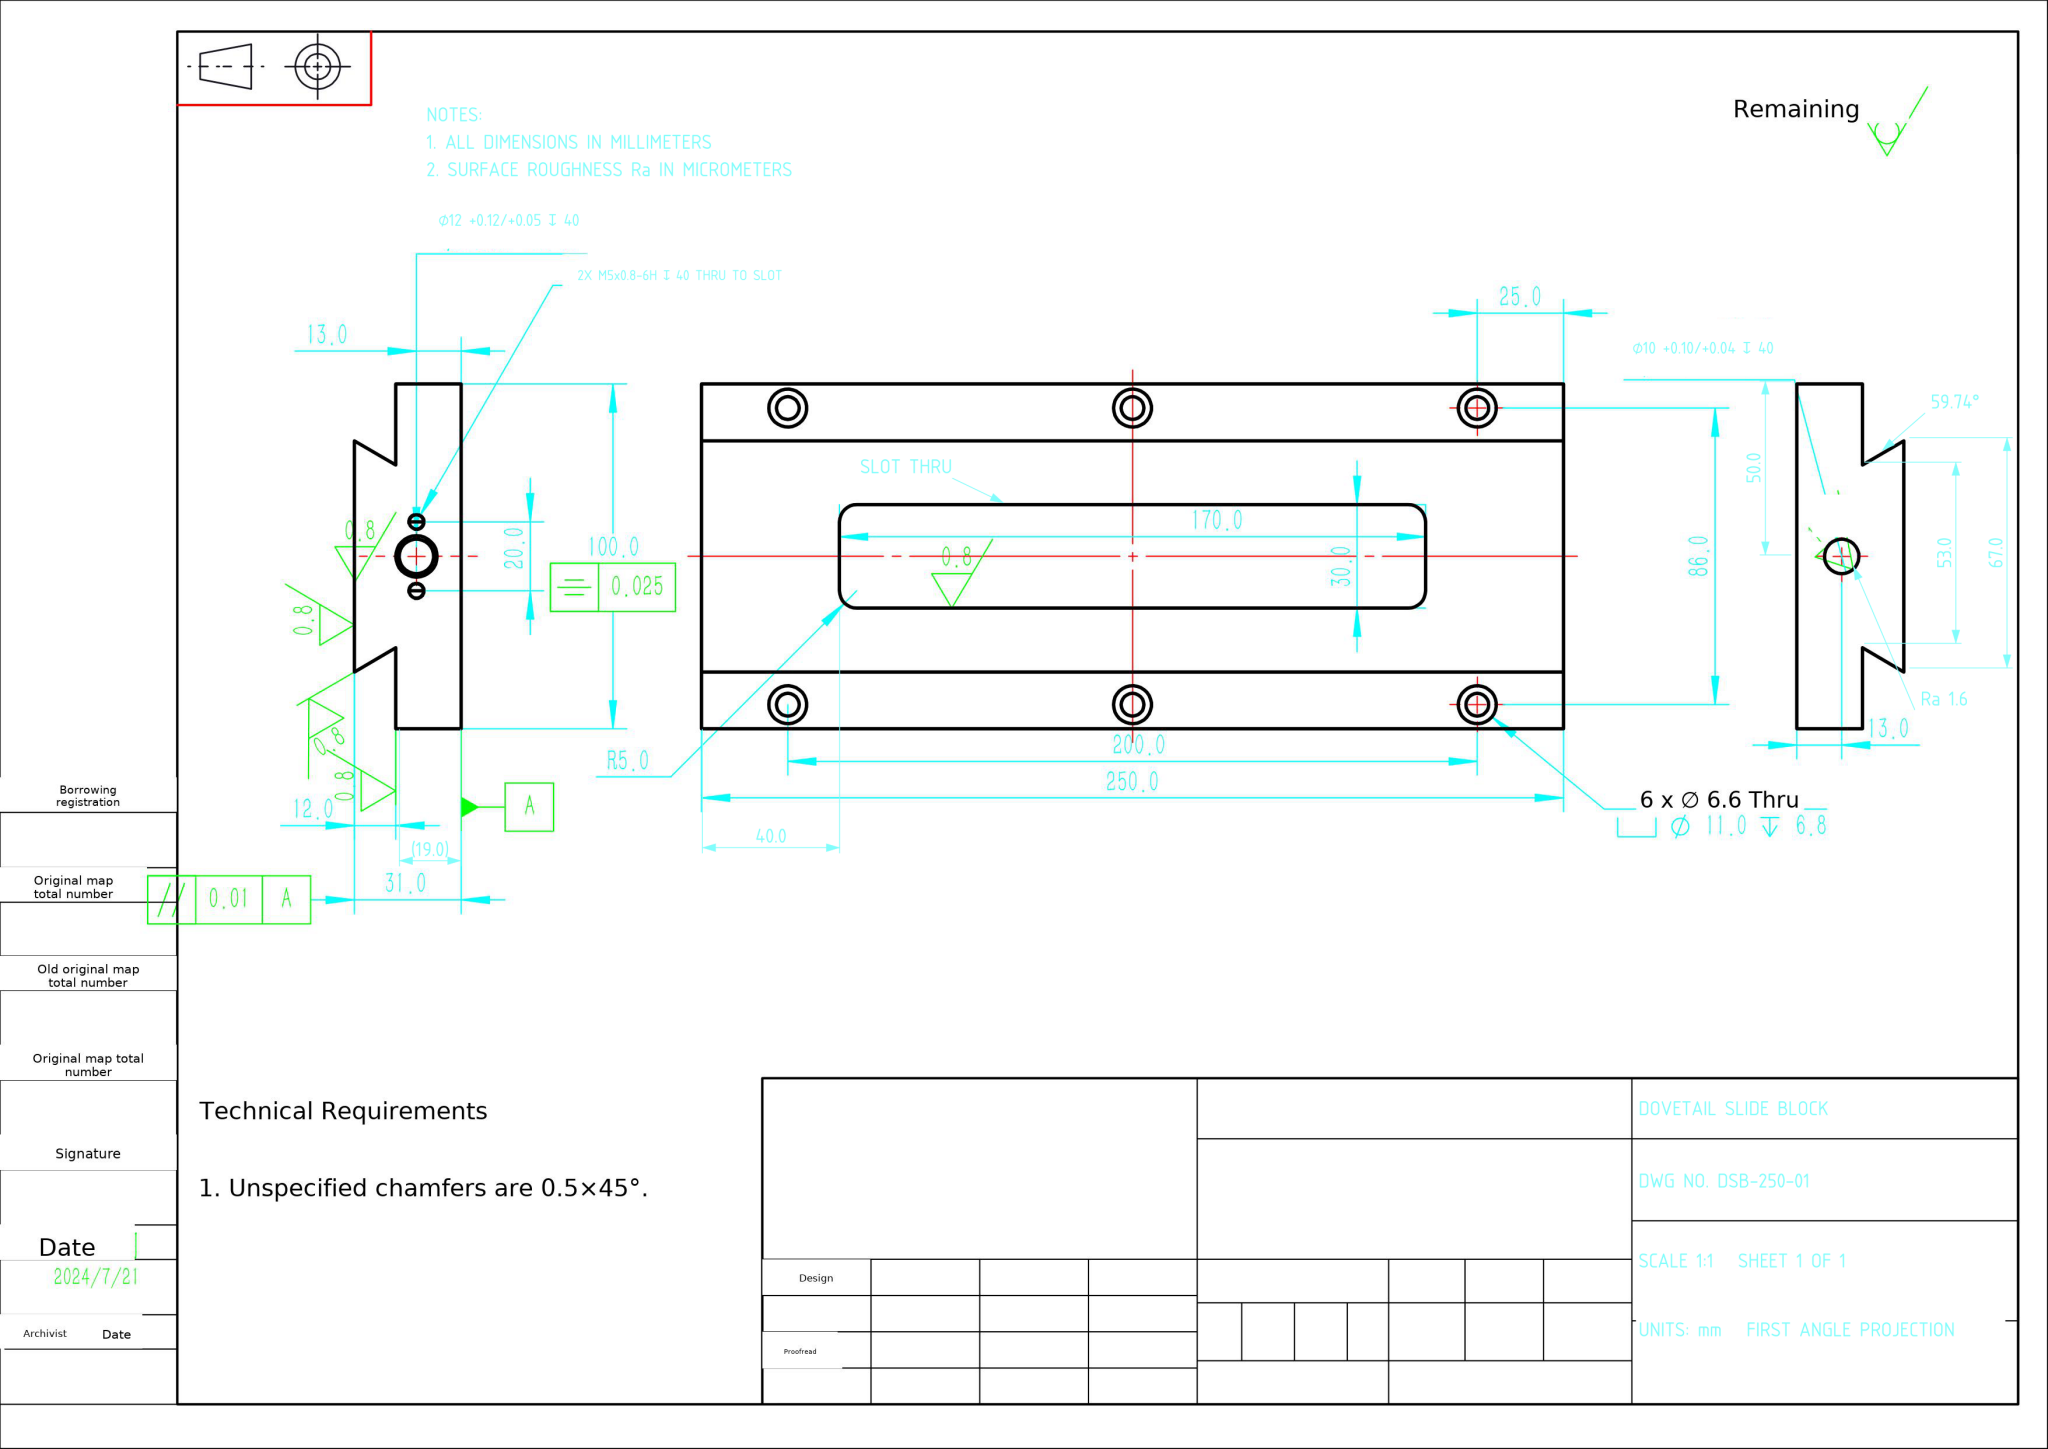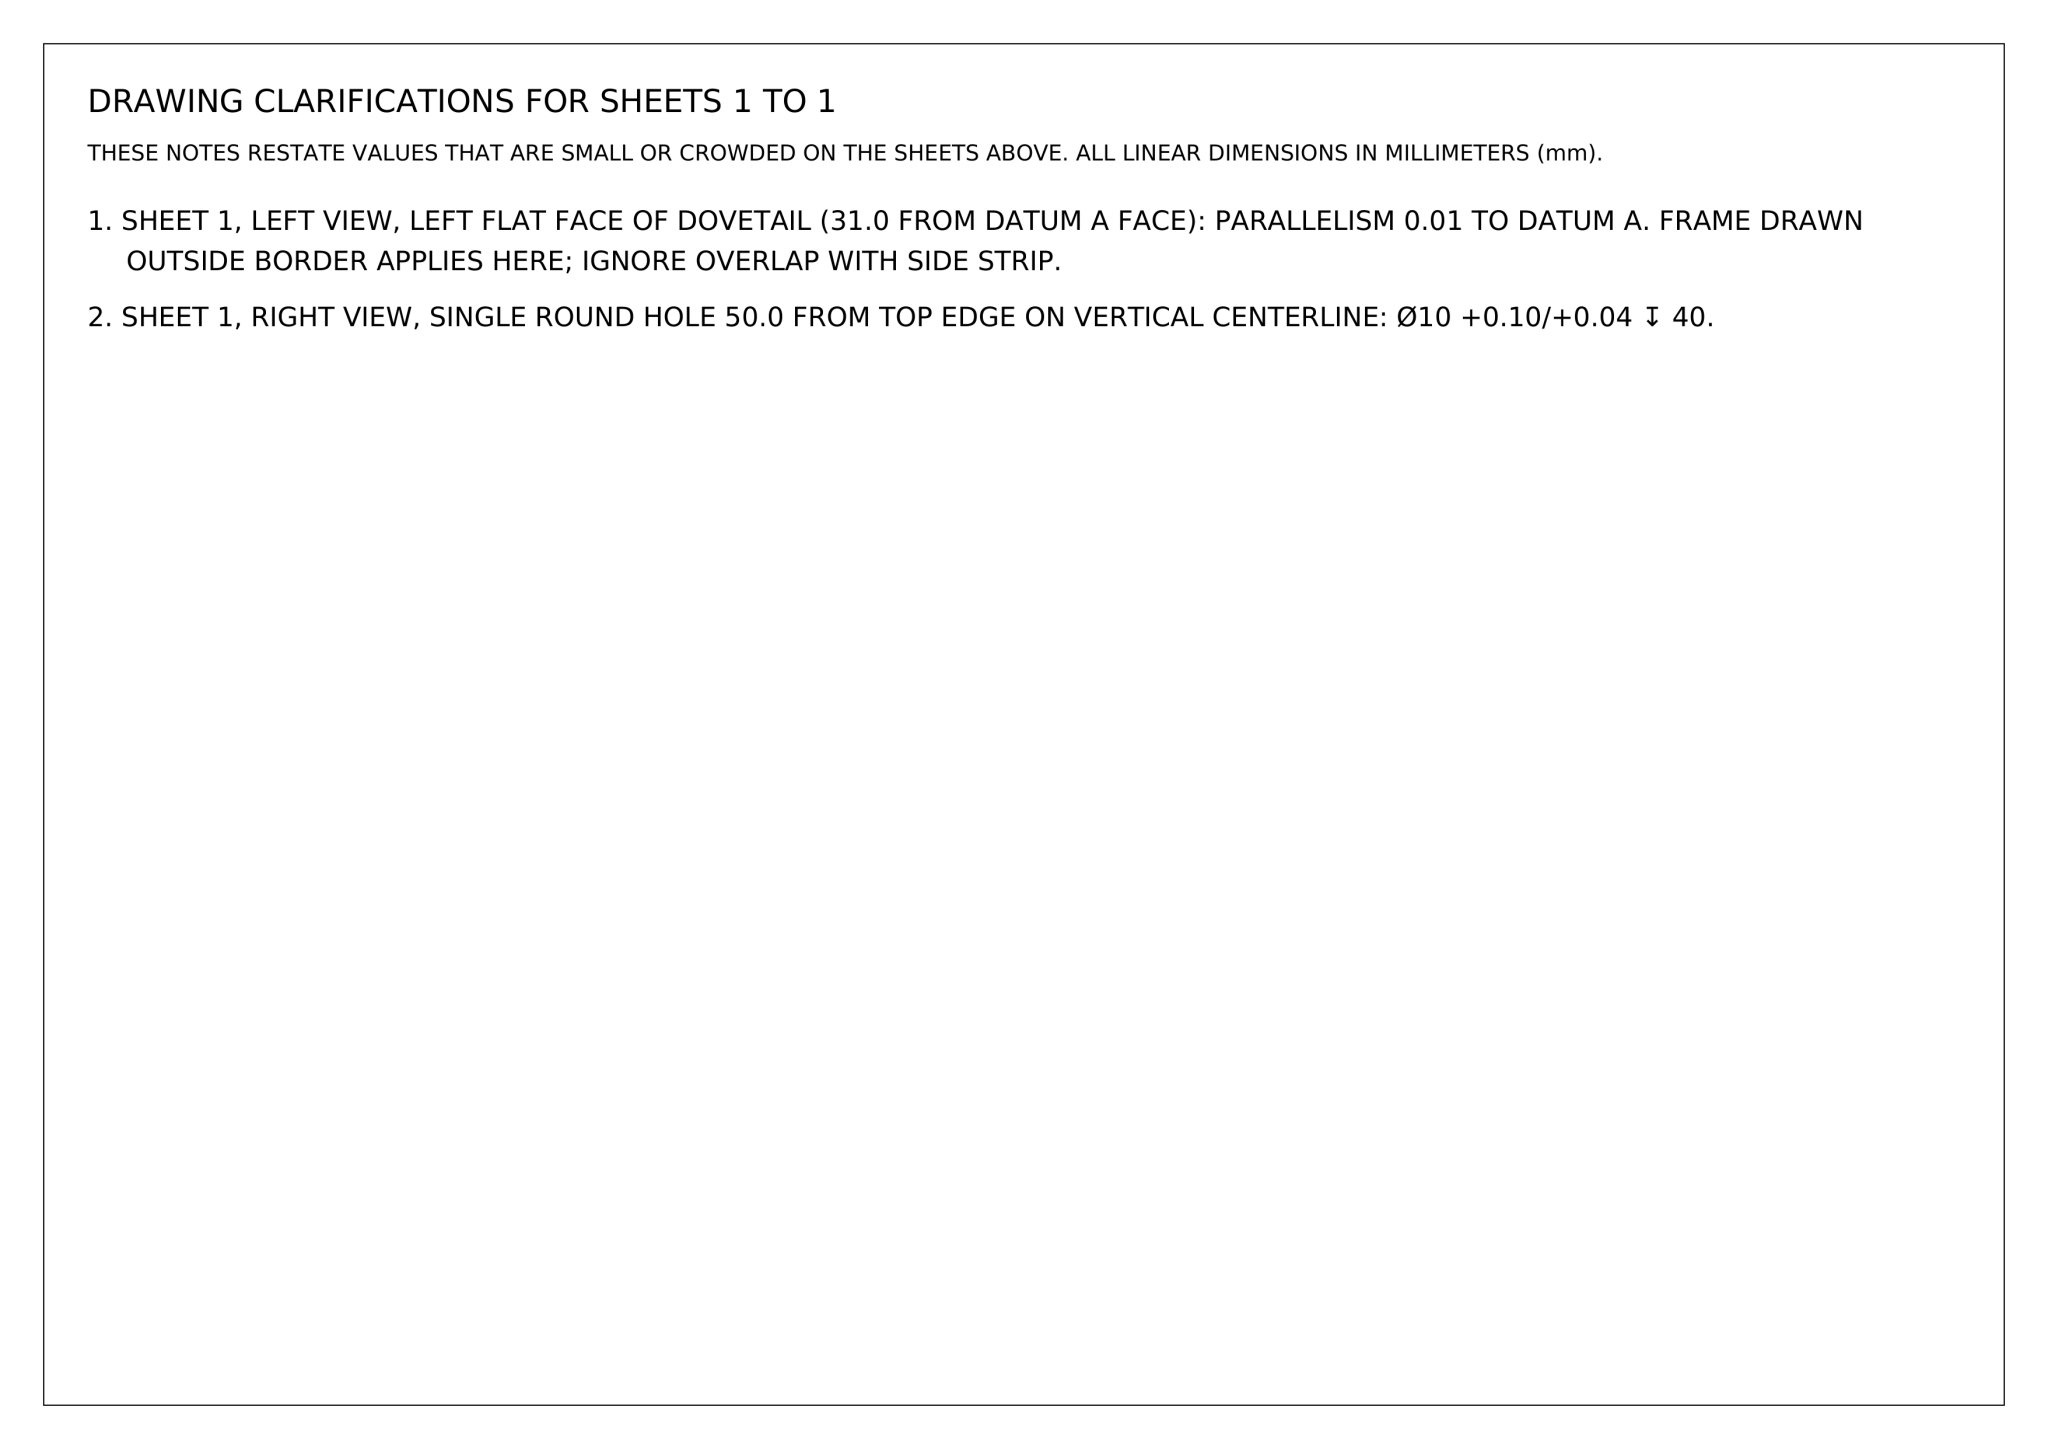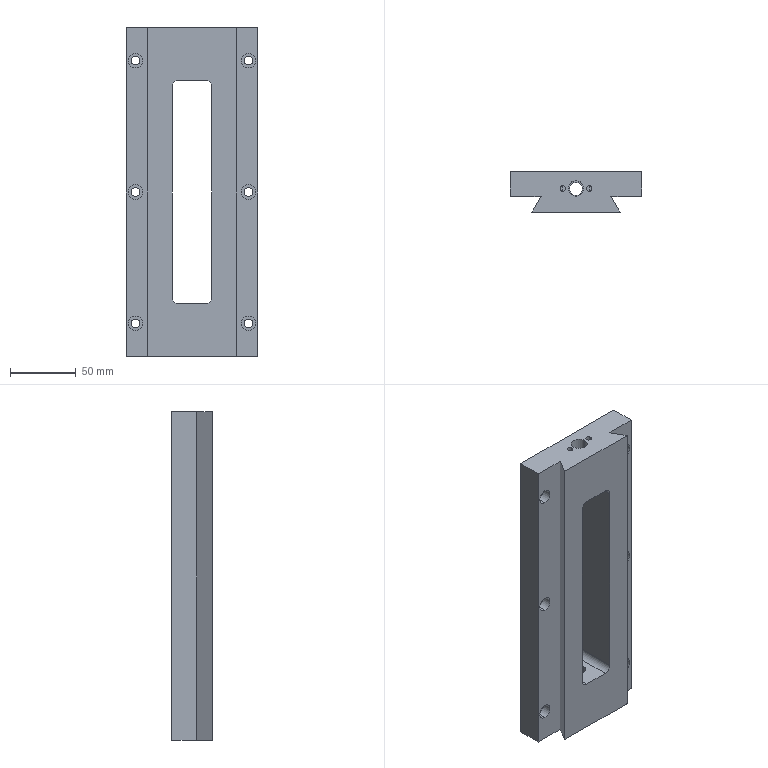Part | NX | mm | 1 solid | 58 faces | box 100 x 31 x 250 mm | volume 482410 mm3 | cylinder 36 | plane 22 | commonest cylinder face diameters 11 x12 6.6 x12 10 x6 4.2 x4 12 x2